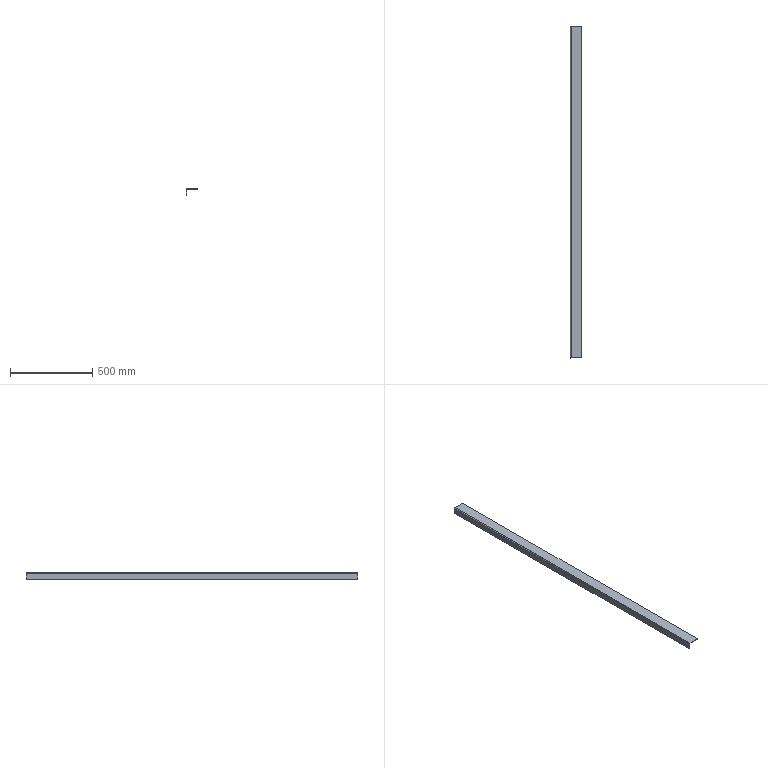Component | SolidWorks | PanelMountingBracket-1 | 1 solid | 14 faces | box 70 x 2020 x 40 mm | volume 428517 mm3 | plane 12 | cylinder 2 | commonest cylinder face diameters 7 x1 11 x1 | material Malleable Cast Iron
STEP:
#1=CARTESIAN_POINT('',(-18.939,76.239,13.07));
#2=VERTEX_POINT('',#1);
#3=CARTESIAN_POINT('',(-18.861,76.239,13.07));
#4=VERTEX_POINT('',#3);
#5=CARTESIAN_POINT('',(-18.939,76.239,13.07));
#6=DIRECTION('',(1.,0.,0.));
#7=VECTOR('',#6,39.37);
#8=LINE('',#5,#7);
#9=EDGE_CURVE('',#2,#4,#8,.T.);
#10=ORIENTED_EDGE('',*,*,#9,.F.);
#11=CARTESIAN_POINT('',(-18.723,76.239,13.286));
#12=VERTEX_POINT('',#11);
#13=CARTESIAN_POINT('',(-18.723,76.239,13.07));
#14=DIRECTION('',(0.,1.,0.));
#15=DIRECTION('',(0.,0.,-1.));
#16=AXIS2_PLACEMENT_3D('',#13,#14,#15);
#17=CIRCLE('',#16,0.2165);
#18=EDGE_CURVE('',#2,#12,#17,.T.);
#19=ORIENTED_EDGE('',*,*,#18,.T.);
#20=CARTESIAN_POINT('',(-18.723,76.239,13.208));
#21=VERTEX_POINT('',#20);
#22=CARTESIAN_POINT('',(-18.723,76.239,13.208));
#23=DIRECTION('',(0.,0.,1.));
#24=VECTOR('',#23,39.37);
#25=LINE('',#22,#24);
#26=EDGE_CURVE('',#21,#12,#25,.T.);
#27=ORIENTED_EDGE('',*,*,#26,.F.);
#28=CARTESIAN_POINT('',(-18.723,76.239,13.07));
#29=DIRECTION('',(0.,1.,0.));
#30=DIRECTION('',(1.,0.,0.));
#31=AXIS2_PLACEMENT_3D('',#28,#29,#30);
#32=CIRCLE('',#31,0.1378);
#33=EDGE_CURVE('',#4,#21,#32,.T.);
#34=ORIENTED_EDGE('',*,*,#33,.F.);
#35=EDGE_LOOP('',(#10,#19,#27,#34));
#36=FACE_OUTER_BOUND('',#35,.T.);
#37=CARTESIAN_POINT('',(-18.939,76.239,13.07));
#38=DIRECTION('',(0.,1.,0.));
#39=DIRECTION('',(0.,0.,1.));
#40=AXIS2_PLACEMENT_3D('',#37,#38,#39);
#41=PLANE('',#40);
#42=ADVANCED_FACE('',(#36),#41,.T.);
#43=CARTESIAN_POINT('',(-18.939,76.239,11.712));
#44=VERTEX_POINT('',#43);
#45=CARTESIAN_POINT('',(-18.939,76.239,11.712));
#46=DIRECTION('',(0.,0.,1.));
#47=VECTOR('',#46,39.37);
#48=LINE('',#45,#47);
#49=EDGE_CURVE('',#44,#2,#48,.T.);
#50=ORIENTED_EDGE('',*,*,#49,.T.);
#51=ORIENTED_EDGE('',*,*,#9,.T.);
#52=CARTESIAN_POINT('',(-18.861,76.239,11.712));
#53=VERTEX_POINT('',#52);
#54=CARTESIAN_POINT('',(-18.861,76.239,11.712));
#55=DIRECTION('',(0.,0.,1.));
#56=VECTOR('',#55,39.37);
#57=LINE('',#54,#56);
#58=EDGE_CURVE('',#53,#4,#57,.T.);
#59=ORIENTED_EDGE('',*,*,#58,.F.);
#60=CARTESIAN_POINT('',(-18.939,76.239,11.712));
#61=DIRECTION('',(1.,0.,0.));
#62=VECTOR('',#61,39.37);
#63=LINE('',#60,#62);
#64=EDGE_CURVE('',#44,#53,#63,.T.);
#65=ORIENTED_EDGE('',*,*,#64,.F.);
#66=EDGE_LOOP('',(#50,#51,#59,#65));
#67=FACE_OUTER_BOUND('',#66,.T.);
#68=CARTESIAN_POINT('',(-18.723,76.239,13.208));
#69=DIRECTION('',(0.,1.,0.));
#70=DIRECTION('',(0.,0.,1.));
#71=AXIS2_PLACEMENT_3D('',#68,#69,#70);
#72=PLANE('',#71);
#73=ADVANCED_FACE('',(#67),#72,.T.);
#74=CARTESIAN_POINT('',(-18.723,-3.289,13.286));
#75=VERTEX_POINT('',#74);
#76=CARTESIAN_POINT('',(-18.723,-3.289,13.208));
#77=VERTEX_POINT('',#76);
#78=CARTESIAN_POINT('',(-18.723,-3.289,13.286));
#79=DIRECTION('',(0.,0.,-1.));
#80=VECTOR('',#79,39.37);
#81=LINE('',#78,#80);
#82=EDGE_CURVE('',#75,#77,#81,.T.);
#83=ORIENTED_EDGE('',*,*,#82,.F.);
#84=CARTESIAN_POINT('',(-18.939,-3.289,13.07));
#85=VERTEX_POINT('',#84);
#86=CARTESIAN_POINT('',(-18.723,-3.289,13.07));
#87=DIRECTION('',(0.,1.,0.));
#88=DIRECTION('',(0.,0.,-1.));
#89=AXIS2_PLACEMENT_3D('',#86,#87,#88);
#90=CIRCLE('',#89,0.2165);
#91=EDGE_CURVE('',#85,#75,#90,.T.);
#92=ORIENTED_EDGE('',*,*,#91,.F.);
#93=CARTESIAN_POINT('',(-18.861,-3.289,13.07));
#94=VERTEX_POINT('',#93);
#95=CARTESIAN_POINT('',(-18.861,-3.289,13.07));
#96=DIRECTION('',(-1.,0.,0.));
#97=VECTOR('',#96,39.37);
#98=LINE('',#95,#97);
#99=EDGE_CURVE('',#94,#85,#98,.T.);
#100=ORIENTED_EDGE('',*,*,#99,.F.);
#101=CARTESIAN_POINT('',(-18.723,-3.289,13.07));
#102=DIRECTION('',(0.,1.,0.));
#103=DIRECTION('',(1.,0.,0.));
#104=AXIS2_PLACEMENT_3D('',#101,#102,#103);
#105=CIRCLE('',#104,0.1378);
#106=EDGE_CURVE('',#94,#77,#105,.T.);
#107=ORIENTED_EDGE('',*,*,#106,.T.);
#108=EDGE_LOOP('',(#83,#92,#100,#107));
#109=FACE_OUTER_BOUND('',#108,.T.);
#110=CARTESIAN_POINT('',(-18.723,-3.289,13.286));
#111=DIRECTION('',(0.,-1.,0.));
#112=DIRECTION('',(0.,0.,-1.));
#113=AXIS2_PLACEMENT_3D('',#110,#111,#112);
#114=PLANE('',#113);
#115=ADVANCED_FACE('',(#109),#114,.T.);
#116=CARTESIAN_POINT('',(-16.183,-3.289,13.286));
#117=VERTEX_POINT('',#116);
#118=CARTESIAN_POINT('',(-18.939,-3.289,13.286));
#119=DIRECTION('',(1.,0.,0.));
#120=VECTOR('',#119,39.37);
#121=LINE('',#118,#120);
#122=EDGE_CURVE('',#75,#117,#121,.T.);
#123=ORIENTED_EDGE('',*,*,#122,.F.);
#124=ORIENTED_EDGE('',*,*,#82,.T.);
#125=CARTESIAN_POINT('',(-16.183,-3.289,13.208));
#126=VERTEX_POINT('',#125);
#127=CARTESIAN_POINT('',(-18.939,-3.289,13.208));
#128=DIRECTION('',(1.,0.,0.));
#129=VECTOR('',#128,39.37);
#130=LINE('',#127,#129);
#131=EDGE_CURVE('',#77,#126,#130,.T.);
#132=ORIENTED_EDGE('',*,*,#131,.T.);
#133=CARTESIAN_POINT('',(-16.183,-3.289,13.208));
#134=DIRECTION('',(0.,0.,1.));
#135=VECTOR('',#134,39.37);
#136=LINE('',#133,#135);
#137=EDGE_CURVE('',#126,#117,#136,.T.);
#138=ORIENTED_EDGE('',*,*,#137,.T.);
#139=EDGE_LOOP('',(#123,#124,#132,#138));
#140=FACE_OUTER_BOUND('',#139,.T.);
#141=CARTESIAN_POINT('',(-18.861,-3.289,13.07));
#142=DIRECTION('',(0.,-1.,0.));
#143=DIRECTION('',(0.,0.,-1.));
#144=AXIS2_PLACEMENT_3D('',#141,#142,#143);
#145=PLANE('',#144);
#146=ADVANCED_FACE('',(#140),#145,.T.);
#147=ORIENTED_EDGE('',*,*,#122,.T.);
#148=CARTESIAN_POINT('',(-16.183,76.239,13.286));
#149=VERTEX_POINT('',#148);
#150=CARTESIAN_POINT('',(-16.183,76.239,13.286));
#151=DIRECTION('',(0.,-1.,0.));
#152=VECTOR('',#151,39.37);
#153=LINE('',#150,#152);
#154=EDGE_CURVE('',#149,#117,#153,.T.);
#155=ORIENTED_EDGE('',*,*,#154,.F.);
#156=CARTESIAN_POINT('',(-18.939,76.239,13.286));
#157=DIRECTION('',(1.,0.,0.));
#158=VECTOR('',#157,39.37);
#159=LINE('',#156,#158);
#160=EDGE_CURVE('',#12,#149,#159,.T.);
#161=ORIENTED_EDGE('',*,*,#160,.F.);
#162=CARTESIAN_POINT('',(-18.723,76.239,13.286));
#163=DIRECTION('',(0.,-1.,0.));
#164=VECTOR('',#163,39.37);
#165=LINE('',#162,#164);
#166=EDGE_CURVE('',#12,#75,#165,.T.);
#167=ORIENTED_EDGE('',*,*,#166,.T.);
#168=EDGE_LOOP('',(#147,#155,#161,#167));
#169=FACE_OUTER_BOUND('',#168,.T.);
#170=CARTESIAN_POINT('',(-18.939,76.239,13.286));
#171=DIRECTION('',(0.,0.,-1.));
#172=DIRECTION('',(-1.,0.,0.));
#173=AXIS2_PLACEMENT_3D('',#170,#171,#172);
#174=PLANE('',#173);
#175=ADVANCED_FACE('',(#169),#174,.F.);
#176=ORIENTED_EDGE('',*,*,#137,.F.);
#177=CARTESIAN_POINT('',(-16.183,76.239,13.208));
#178=VERTEX_POINT('',#177);
#179=CARTESIAN_POINT('',(-16.183,76.239,13.208));
#180=DIRECTION('',(0.,-1.,0.));
#181=VECTOR('',#180,39.37);
#182=LINE('',#179,#181);
#183=EDGE_CURVE('',#178,#126,#182,.T.);
#184=ORIENTED_EDGE('',*,*,#183,.F.);
#185=CARTESIAN_POINT('',(-16.183,76.239,13.208));
#186=DIRECTION('',(0.,0.,1.));
#187=VECTOR('',#186,39.37);
#188=LINE('',#185,#187);
#189=EDGE_CURVE('',#178,#149,#188,.T.);
#190=ORIENTED_EDGE('',*,*,#189,.T.);
#191=ORIENTED_EDGE('',*,*,#154,.T.);
#192=EDGE_LOOP('',(#176,#184,#190,#191));
#193=FACE_OUTER_BOUND('',#192,.T.);
#194=CARTESIAN_POINT('',(-16.183,76.239,13.208));
#195=DIRECTION('',(1.,0.,0.));
#196=DIRECTION('',(0.,0.,-1.));
#197=AXIS2_PLACEMENT_3D('',#194,#195,#196);
#198=PLANE('',#197);
#199=ADVANCED_FACE('',(#193),#198,.T.);
#200=ORIENTED_EDGE('',*,*,#131,.F.);
#201=CARTESIAN_POINT('',(-18.723,76.239,13.208));
#202=DIRECTION('',(0.,-1.,0.));
#203=VECTOR('',#202,39.37);
#204=LINE('',#201,#203);
#205=EDGE_CURVE('',#21,#77,#204,.T.);
#206=ORIENTED_EDGE('',*,*,#205,.F.);
#207=CARTESIAN_POINT('',(-18.939,76.239,13.208));
#208=DIRECTION('',(1.,0.,0.));
#209=VECTOR('',#208,39.37);
#210=LINE('',#207,#209);
#211=EDGE_CURVE('',#21,#178,#210,.T.);
#212=ORIENTED_EDGE('',*,*,#211,.T.);
#213=ORIENTED_EDGE('',*,*,#183,.T.);
#214=EDGE_LOOP('',(#200,#206,#212,#213));
#215=FACE_OUTER_BOUND('',#214,.T.);
#216=CARTESIAN_POINT('',(-18.939,76.239,13.208));
#217=DIRECTION('',(0.,0.,-1.));
#218=DIRECTION('',(-1.,0.,0.));
#219=AXIS2_PLACEMENT_3D('',#216,#217,#218);
#220=PLANE('',#219);
#221=ADVANCED_FACE('',(#215),#220,.T.);
#222=ORIENTED_EDGE('',*,*,#106,.F.);
#223=CARTESIAN_POINT('',(-18.861,76.239,13.07));
#224=DIRECTION('',(0.,-1.,0.));
#225=VECTOR('',#224,39.37);
#226=LINE('',#223,#225);
#227=EDGE_CURVE('',#4,#94,#226,.T.);
#228=ORIENTED_EDGE('',*,*,#227,.F.);
#229=ORIENTED_EDGE('',*,*,#33,.T.);
#230=ORIENTED_EDGE('',*,*,#205,.T.);
#231=EDGE_LOOP('',(#222,#228,#229,#230));
#232=FACE_OUTER_BOUND('',#231,.T.);
#233=CARTESIAN_POINT('',(-18.723,76.239,13.07));
#234=DIRECTION('',(0.,-1.,0.));
#235=DIRECTION('',(0.,0.,-1.));
#236=AXIS2_PLACEMENT_3D('',#233,#234,#235);
#237=CYLINDRICAL_SURFACE('',#236,0.1378);
#238=ADVANCED_FACE('',(#232),#237,.F.);
#239=CARTESIAN_POINT('',(-18.861,-3.289,11.712));
#240=VERTEX_POINT('',#239);
#241=CARTESIAN_POINT('',(-18.861,-3.289,11.712));
#242=DIRECTION('',(0.,0.,1.));
#243=VECTOR('',#242,39.37);
#244=LINE('',#241,#243);
#245=EDGE_CURVE('',#240,#94,#244,.T.);
#246=ORIENTED_EDGE('',*,*,#245,.F.);
#247=CARTESIAN_POINT('',(-18.861,76.239,11.712));
#248=DIRECTION('',(0.,-1.,0.));
#249=VECTOR('',#248,39.37);
#250=LINE('',#247,#249);
#251=EDGE_CURVE('',#53,#240,#250,.T.);
#252=ORIENTED_EDGE('',*,*,#251,.F.);
#253=ORIENTED_EDGE('',*,*,#58,.T.);
#254=ORIENTED_EDGE('',*,*,#227,.T.);
#255=EDGE_LOOP('',(#246,#252,#253,#254));
#256=FACE_OUTER_BOUND('',#255,.T.);
#257=CARTESIAN_POINT('',(-18.861,76.239,11.712));
#258=DIRECTION('',(1.,0.,0.));
#259=DIRECTION('',(0.,0.,-1.));
#260=AXIS2_PLACEMENT_3D('',#257,#258,#259);
#261=PLANE('',#260);
#262=ADVANCED_FACE('',(#256),#261,.T.);
#263=CARTESIAN_POINT('',(-18.939,-3.289,11.712));
#264=VERTEX_POINT('',#263);
#265=CARTESIAN_POINT('',(-18.939,-3.289,11.712));
#266=DIRECTION('',(1.,0.,0.));
#267=VECTOR('',#266,39.37);
#268=LINE('',#265,#267);
#269=EDGE_CURVE('',#264,#240,#268,.T.);
#270=ORIENTED_EDGE('',*,*,#269,.F.);
#271=CARTESIAN_POINT('',(-18.939,76.239,11.712));
#272=DIRECTION('',(0.,-1.,0.));
#273=VECTOR('',#272,39.37);
#274=LINE('',#271,#273);
#275=EDGE_CURVE('',#44,#264,#274,.T.);
#276=ORIENTED_EDGE('',*,*,#275,.F.);
#277=ORIENTED_EDGE('',*,*,#64,.T.);
#278=ORIENTED_EDGE('',*,*,#251,.T.);
#279=EDGE_LOOP('',(#270,#276,#277,#278));
#280=FACE_OUTER_BOUND('',#279,.T.);
#281=CARTESIAN_POINT('',(-18.939,76.239,11.712));
#282=DIRECTION('',(0.,0.,-1.));
#283=DIRECTION('',(-1.,0.,0.));
#284=AXIS2_PLACEMENT_3D('',#281,#282,#283);
#285=PLANE('',#284);
#286=ADVANCED_FACE('',(#280),#285,.T.);
#287=CARTESIAN_POINT('',(-18.939,-3.289,11.712));
#288=DIRECTION('',(0.,0.,1.));
#289=VECTOR('',#288,39.37);
#290=LINE('',#287,#289);
#291=EDGE_CURVE('',#264,#85,#290,.T.);
#292=ORIENTED_EDGE('',*,*,#291,.T.);
#293=CARTESIAN_POINT('',(-18.939,76.239,13.07));
#294=DIRECTION('',(0.,-1.,0.));
#295=VECTOR('',#294,39.37);
#296=LINE('',#293,#295);
#297=EDGE_CURVE('',#2,#85,#296,.T.);
#298=ORIENTED_EDGE('',*,*,#297,.F.);
#299=ORIENTED_EDGE('',*,*,#49,.F.);
#300=ORIENTED_EDGE('',*,*,#275,.T.);
#301=EDGE_LOOP('',(#292,#298,#299,#300));
#302=FACE_OUTER_BOUND('',#301,.T.);
#303=CARTESIAN_POINT('',(-18.939,76.239,11.712));
#304=DIRECTION('',(1.,0.,0.));
#305=DIRECTION('',(0.,0.,-1.));
#306=AXIS2_PLACEMENT_3D('',#303,#304,#305);
#307=PLANE('',#306);
#308=ADVANCED_FACE('',(#302),#307,.F.);
#309=ORIENTED_EDGE('',*,*,#91,.T.);
#310=ORIENTED_EDGE('',*,*,#166,.F.);
#311=ORIENTED_EDGE('',*,*,#18,.F.);
#312=ORIENTED_EDGE('',*,*,#297,.T.);
#313=EDGE_LOOP('',(#309,#310,#311,#312));
#314=FACE_OUTER_BOUND('',#313,.T.);
#315=CARTESIAN_POINT('',(-18.723,76.239,13.07));
#316=DIRECTION('',(0.,-1.,0.));
#317=DIRECTION('',(0.,0.,-1.));
#318=AXIS2_PLACEMENT_3D('',#315,#316,#317);
#319=CYLINDRICAL_SURFACE('',#318,0.2165);
#320=ADVANCED_FACE('',(#314),#319,.T.);
#321=ORIENTED_EDGE('',*,*,#160,.T.);
#322=ORIENTED_EDGE('',*,*,#189,.F.);
#323=ORIENTED_EDGE('',*,*,#211,.F.);
#324=ORIENTED_EDGE('',*,*,#26,.T.);
#325=EDGE_LOOP('',(#321,#322,#323,#324));
#326=FACE_OUTER_BOUND('',#325,.T.);
#327=CARTESIAN_POINT('',(-18.723,76.239,13.07));
#328=DIRECTION('',(0.,1.,0.));
#329=DIRECTION('',(1.,0.,0.));
#330=AXIS2_PLACEMENT_3D('',#327,#328,#329);
#331=PLANE('',#330);
#332=ADVANCED_FACE('',(#326),#331,.T.);
#333=ORIENTED_EDGE('',*,*,#245,.T.);
#334=ORIENTED_EDGE('',*,*,#99,.T.);
#335=ORIENTED_EDGE('',*,*,#291,.F.);
#336=ORIENTED_EDGE('',*,*,#269,.T.);
#337=EDGE_LOOP('',(#333,#334,#335,#336));
#338=FACE_OUTER_BOUND('',#337,.T.);
#339=CARTESIAN_POINT('',(-18.723,-3.289,13.07));
#340=DIRECTION('',(0.,1.,0.));
#341=DIRECTION('',(1.,0.,0.));
#342=AXIS2_PLACEMENT_3D('',#339,#340,#341);
#343=PLANE('',#342);
#344=ADVANCED_FACE('',(#338),#343,.F.);
#345=CLOSED_SHELL('',(#42,#73,#115,#146,#175,#199,#221,#238,#262,#286,#308,#320,#332,#344));
#346=MANIFOLD_SOLID_BREP('',#345);
#347=CARTESIAN_POINT('',(0.,0.,0.));
#348=DIRECTION('',(0.,0.,1.));
#349=DIRECTION('',(1.,0.,0.));
#350=AXIS2_PLACEMENT_3D('',#347,#348,#349);
#351=(LENGTH_UNIT()NAMED_UNIT(*)SI_UNIT($,.METRE.));
#352=LENGTH_MEASURE_WITH_UNIT(LENGTH_MEASURE(0.0254),#351);
#353=DIMENSIONAL_EXPONENTS(1.,0.,0.,0.,0.,0.,0.);
#354=(CONVERSION_BASED_UNIT('',#352)LENGTH_UNIT()NAMED_UNIT(#353));
#355=UNCERTAINTY_MEASURE_WITH_UNIT(LENGTH_MEASURE(0.00001),#354,'','');
#356=(NAMED_UNIT(*)PLANE_ANGLE_UNIT()SI_UNIT($,.RADIAN.));
#357=(NAMED_UNIT(*)SI_UNIT($,.STERADIAN.)SOLID_ANGLE_UNIT());
#358=(GEOMETRIC_REPRESENTATION_CONTEXT(3)GLOBAL_UNCERTAINTY_ASSIGNED_CONTEXT((#355))GLOBAL_UNIT_ASSIGNED_CONTEXT((#354,#356,#357))REPRESENTATION_CONTEXT('',''));
#359=ADVANCED_BREP_SHAPE_REPRESENTATION('',(#346,#350),#358);
#360=COLOUR_RGB('',0.7922,0.8196,0.9333);
#361=FILL_AREA_STYLE_COLOUR('',#360);
#362=FILL_AREA_STYLE('',(#361));
#363=SURFACE_STYLE_FILL_AREA(#362);
#364=SURFACE_SIDE_STYLE('',(#363));
#365=SURFACE_STYLE_USAGE(.BOTH.,#364);
#366=PRESENTATION_STYLE_ASSIGNMENT((#365));
#367=STYLED_ITEM('',(#366),#346);
#368=PRESENTATION_LAYER_ASSIGNMENT('','',(#367));
#369=(LENGTH_UNIT()NAMED_UNIT(*)SI_UNIT($,.METRE.));
#370=LENGTH_MEASURE_WITH_UNIT(LENGTH_MEASURE(0.0254),#369);
#371=DIMENSIONAL_EXPONENTS(1.,0.,0.,0.,0.,0.,0.);
#372=(CONVERSION_BASED_UNIT('',#370)LENGTH_UNIT()NAMED_UNIT(#371));
#373=UNCERTAINTY_MEASURE_WITH_UNIT(LENGTH_MEASURE(0.00001),#372,'','');
#374=(NAMED_UNIT(*)PLANE_ANGLE_UNIT()SI_UNIT($,.RADIAN.));
#375=(NAMED_UNIT(*)SI_UNIT($,.STERADIAN.)SOLID_ANGLE_UNIT());
#376=(GEOMETRIC_REPRESENTATION_CONTEXT(3)GLOBAL_UNCERTAINTY_ASSIGNED_CONTEXT((#373))GLOBAL_UNIT_ASSIGNED_CONTEXT((#372,#374,#375))REPRESENTATION_CONTEXT('',''));
#377=MECHANICAL_DESIGN_GEOMETRIC_PRESENTATION_REPRESENTATION('',(#367),#376);